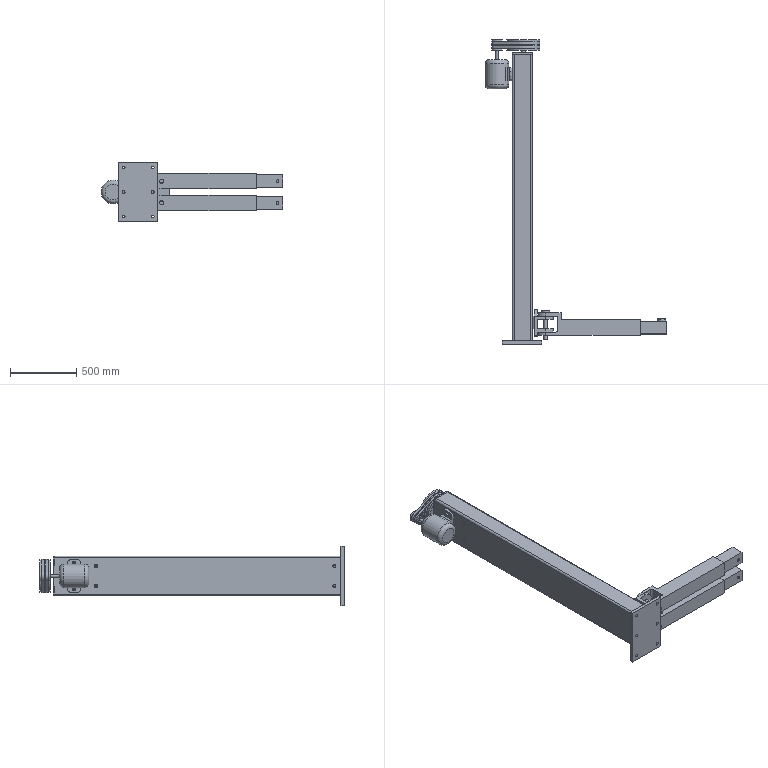Assembly | NX | mm | 19 component files | 21 solids | 358 faces | box 1374 x 2300 x 450 mm | volume 4471591 mm3 | plane 208 | cylinder 106 | cone 24 | spline 14 | torus 6 | commonest cylinder face diameters 30 x14 28 x12 25 x11 116 x8 20 x8 60 x8 22 x7 80 x6
Bill of materials:
unnamed part 1 | 1 |  | Short, wide disc that turns about one axis. Two V-shaped grooves run around its rim, and it has a small central bore with a keyway notch. A shallow circular recess is cut into the face, just inside the outer rim.
unnamed part 2 | 1 |  | Cylinder with rounded edges, with a rounded-rectangle mounting tab joined to one side by a short tapered neck. The tab has two through-holes, one near each end.
unnamed part 3 | 1 |  | Cylindrical head with rounded edges and a long, thin round rod coming out of the centre of one end.
unnamed part 4 | 1 |  | Very long, slender round rod. Most of its length has closely spaced ridges, and both ends have short plain sections; one plain end is longer and stepped smaller.
unnamed part 5 | 2 |  | Straight, thin-walled hollow tube with a square cross-section and open ends. A cylindrical rod runs across the inside near one end, and there is a small round hole in a side wall near the same end.
unnamed part 6 | 1 |  | Plate-type bracket. A main plate has a profile with one pointed rounded lobe and one rounded-rectangle end. It has one hole in the lobe and two holes at the rounded end. Two parallel plates stand out from it, each with two holes.
unnamed part 7 | 2 |  | Long hollow tube arm with a rectangular cross-section and an open end. The other end has a fork made of two parallel lugs with rounded ends, each with a through-hole on the same axis.
unnamed part 8 | 1 |  | Long beam with a channel-like (C-shaped) cross-section, attached to a rectangular end plate at one end. The plate has six holes in two columns of three. The beam web has a few small holes, and there is a cutout near the far end.
unnamed part 9 | 2 |  | Headed pin with a plain round shaft and a larger round head. The rim of the head has four rectangular notches around it.
unnamed part 10 | 2 |  | Thin, closed teardrop-shaped loop. One end is a large rounded arc and the other a small rounded arc, joined by two straight tangent sides. The band has a narrow rectangular cross-section.
unnamed part 11 | 2 |  | Simple headed pin: a plain round shaft with a short, flat, round head of larger diameter on one end.
unnamed part 12 | 1 |  | Round grooved hub with two V-shaped grooves around its outside, and a fairly large central bore with a keyway notch. One face has a recessed area inside the outer ring.
unnamed part 13 | 2 |  | Single-piece tab/lug bracket: a flat rectangular base plate with one through hole near each end. A single tab sticks out at a right angle from the middle of the plate. The tab has the same width as the plate, a semicircular rounded end, and one through hole on the same center as that rounded end. Where the tab meets the plate, the corners have fillets.
Mates:
1. center | motor_mount 1 | motor_mount 1 | motor_rotor 1 | motor_rotor 1
2. touch align | motor_rotor 1 | motor_mount 1
3. touch align | motor_mount 1 | assembly datumaxis
4. center | lead_screw_mount 2 face | lead_screw_mount 2 face | column 1
5. touch align | lead_screw_mount 2 face | column 1 face
6. distance | lead_screw_mount 2 face | column 1 face
7. fix | assembly component
8. bond | lead_screw_mount 2 component | assembly component
9. bond | lead_screw_mount 1 component | assembly component
10. linear | assembly datumaxis | assembly cartesiancoordinatesystem | assembly cartesiancoordinatesystem
11. touch align | moving_block 1 face | lead_screw_mount 2 face
12. parallel | moving_block 1 | column 1 face
13. concentric | swing_rod 2 edge | moving_block 1 edge
14. concentric | swing_rod 1 edge | moving_block 1 edge
15. center | telescopic_rod 2 face | telescopic_rod 2 face | swing_rod 2 face | swing_rod 2 face
16. center | telescopic_rod 2 face | telescopic_rod 2 face | swing_rod 2 face | swing_rod 2 face
17. center | telescopic_rod 1 face | telescopic_rod 1 face | swing_rod 1 face | swing_rod 1 face
18. center | telescopic_rod 1 face | telescopic_rod 1 face | swing_rod 1 face | swing_rod 1 face
19. distance | telescopic_rod 2 face | swing_rod 2 face
20. distance | telescopic_rod 1 face | swing_rod 1 face
21. concentric | driven_wheel 1 edge | lead_screw 1 edge
22. touch align | motor 1 face | column 1 face
23. center | motor 1 face | motor 1 face | column 1 face | column 1 face
24. distance | lead_screw 1 face | lead_screw_mount 1 face
25. touch align | motor 1 face | lead_screw 1 face
26. concentric | drive_wheel 1 edge | motor 1 edge
27. touch align | belt 2 | drive_wheel 1 face
28. bond | drive_wheel 1 component | assembly component
29. bond | belt 2 component | assembly component
30. bond | belt 1 component | assembly component
31. linear | assembly datumaxis | assembly cartesiancoordinatesystem | assembly cartesiancoordinatesystem
32. touch align | moving_block 1 face | lead_screw_mount 2 face
33. touch align | pin 2 face | swing_rod 2 face
34. touch align | pin 2 face | swing_rod 2 face
35. touch align | pin 1 face | swing_rod 1 face
36. touch align | pin 1 face | swing_rod 1 face
37. concentric | adjust_screw 1 edge | telescopic_rod 2 edge
38. concentric | adjust_screw 2 edge | telescopic_rod 1 edge